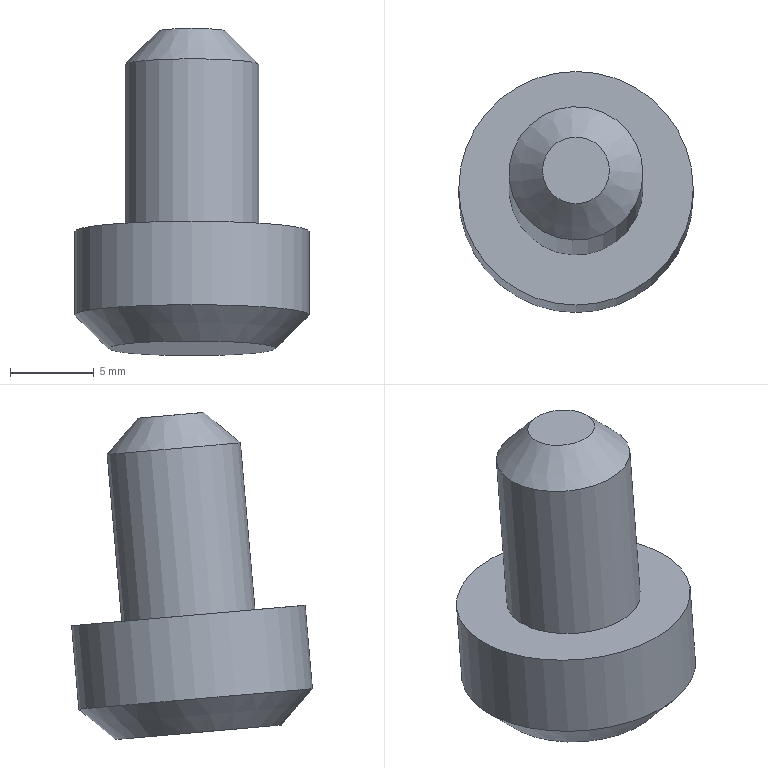Component | NX | BASE_FOOT | 1 solid | 7 faces | box 14 x 14.38 x 19.54 mm | volume 1559 mm3 | plane 3 | cylinder 2 | cone 2 | commonest cylinder face diameters 14 x1 8 x1
STEP:
#1=CARTESIAN_POINT('',(0.,0.,0.));
#2=DIRECTION('',(0.,0.,1.));
#3=DIRECTION('',(1.,0.,0.));
#4=AXIS2_PLACEMENT_3D('',#1,#2,#3);
#5=CARTESIAN_POINT('',(402.941,512.422,-69.71));
#6=VERTEX_POINT('',#5);
#7=CARTESIAN_POINT('',(395.941,512.422,-69.71));
#8=DIRECTION('',(0.,0.08716,0.9962));
#9=DIRECTION('',(1.,0.,0.));
#10=AXIS2_PLACEMENT_3D('',#7,#8,#9);
#11=CIRCLE('',#10,7.);
#12=CARTESIAN_POINT('',(395.941,512.858,-64.729));
#13=DIRECTION('',(0.,-0.08716,-0.9962));
#14=DIRECTION('',(-1.,0.,0.));
#15=AXIS2_PLACEMENT_3D('',#12,#13,#14);
#16=CYLINDRICAL_SURFACE('',#15,7.);
#17=CARTESIAN_POINT('',(9.425,5.));
#18=DIRECTION('',(-1.,0.));
#19=VECTOR('',#18,1.);
#20=LINE('',#17,#19);
#21=(GEOMETRIC_REPRESENTATION_CONTEXT(2)PARAMETRIC_REPRESENTATION_CONTEXT()REPRESENTATION_CONTEXT('',''));
#22=DEFINITIONAL_REPRESENTATION('',(#20),#21);
#23=PCURVE('',#16,#22);
#24=CARTESIAN_POINT('',(395.941,512.422,-69.71));
#25=DIRECTION('',(0.,0.08716,0.9962));
#26=DIRECTION('',(1.,0.,-0.));
#27=AXIS2_PLACEMENT_3D('',#24,#25,#26);
#28=CONICAL_SURFACE('',#27,7.,0.7854);
#29=CARTESIAN_POINT('',(0.,0.));
#30=DIRECTION('',(1.,0.));
#31=VECTOR('',#30,1.);
#32=LINE('',#29,#31);
#33=(GEOMETRIC_REPRESENTATION_CONTEXT(2)PARAMETRIC_REPRESENTATION_CONTEXT()REPRESENTATION_CONTEXT('',''));
#34=DEFINITIONAL_REPRESENTATION('',(#32),#33);
#35=PCURVE('',#28,#34);
#36=SURFACE_CURVE('',#11,(#23,#35),.PCURVE_S1.);
#37=EDGE_CURVE('',#6,#6,#36,.T.);
#38=ORIENTED_EDGE('',*,*,#37,.T.);
#39=CARTESIAN_POINT('',(402.941,512.858,-64.729));
#40=VERTEX_POINT('',#39);
#41=CARTESIAN_POINT('',(402.941,512.858,-64.729));
#42=CARTESIAN_POINT('',(402.941,512.422,-69.71));
#43=B_SPLINE_CURVE_WITH_KNOTS('',1,(#41,#42),.UNSPECIFIED.,.F.,.F.,(2,2),(0.,5.),.PIECEWISE_BEZIER_KNOTS.);
#44=CARTESIAN_POINT('',(3.142,0.));
#45=DIRECTION('',(0.,1.));
#46=VECTOR('',#45,1.);
#47=LINE('',#44,#46);
#48=(GEOMETRIC_REPRESENTATION_CONTEXT(2)PARAMETRIC_REPRESENTATION_CONTEXT()REPRESENTATION_CONTEXT('',''));
#49=DEFINITIONAL_REPRESENTATION('',(#47),#48);
#50=PCURVE('',#16,#49);
#51=CARTESIAN_POINT('',(9.425,0.));
#52=DIRECTION('',(0.,1.));
#53=VECTOR('',#52,1.);
#54=LINE('',#51,#53);
#55=(GEOMETRIC_REPRESENTATION_CONTEXT(2)PARAMETRIC_REPRESENTATION_CONTEXT()REPRESENTATION_CONTEXT('',''));
#56=DEFINITIONAL_REPRESENTATION('',(#54),#55);
#57=PCURVE('',#16,#56);
#58=SEAM_CURVE('',#43,(#50,#57),.PCURVE_S1.);
#59=EDGE_CURVE('',#40,#6,#58,.T.);
#60=ORIENTED_EDGE('',*,*,#59,.F.);
#61=CARTESIAN_POINT('',(395.941,512.858,-64.729));
#62=DIRECTION('',(0.,0.08716,0.9962));
#63=DIRECTION('',(1.,0.,0.));
#64=AXIS2_PLACEMENT_3D('',#61,#62,#63);
#65=CIRCLE('',#64,7.);
#66=CARTESIAN_POINT('',(9.425,0.));
#67=DIRECTION('',(-1.,0.));
#68=VECTOR('',#67,1.);
#69=LINE('',#66,#68);
#70=(GEOMETRIC_REPRESENTATION_CONTEXT(2)PARAMETRIC_REPRESENTATION_CONTEXT()REPRESENTATION_CONTEXT('',''));
#71=DEFINITIONAL_REPRESENTATION('',(#69),#70);
#72=PCURVE('',#16,#71);
#73=CARTESIAN_POINT('',(395.941,512.858,-64.729));
#74=DIRECTION('',(0.,0.08716,0.9962));
#75=DIRECTION('',(1.,0.,0.));
#76=AXIS2_PLACEMENT_3D('',#73,#74,#75);
#77=PLANE('',#76);
#78=CARTESIAN_POINT('',(0.,0.));
#79=DIRECTION('',(1.,0.));
#80=AXIS2_PLACEMENT_2D('',#78,#79);
#81=CIRCLE('',#80,7.);
#82=(GEOMETRIC_REPRESENTATION_CONTEXT(2)PARAMETRIC_REPRESENTATION_CONTEXT()REPRESENTATION_CONTEXT('',''));
#83=DEFINITIONAL_REPRESENTATION('',(#81),#82);
#84=PCURVE('',#77,#83);
#85=SURFACE_CURVE('',#65,(#72,#84),.PCURVE_S1.);
#86=EDGE_CURVE('',#40,#40,#85,.T.);
#87=ORIENTED_EDGE('',*,*,#86,.F.);
#88=ORIENTED_EDGE('',*,*,#59,.T.);
#89=EDGE_LOOP('',(#38,#60,#87,#88));
#90=FACE_BOUND('',#89,.T.);
#91=ADVANCED_FACE('',(#90),#16,.T.);
#92=CARTESIAN_POINT('',(399.941,512.858,-64.729));
#93=VERTEX_POINT('',#92);
#94=CARTESIAN_POINT('',(395.941,512.858,-64.729));
#95=DIRECTION('',(0.,0.08716,0.9962));
#96=DIRECTION('',(1.,0.,0.));
#97=AXIS2_PLACEMENT_3D('',#94,#95,#96);
#98=CIRCLE('',#97,4.);
#99=CARTESIAN_POINT('',(0.,0.));
#100=DIRECTION('',(1.,0.));
#101=AXIS2_PLACEMENT_2D('',#99,#100);
#102=CIRCLE('',#101,4.);
#103=(GEOMETRIC_REPRESENTATION_CONTEXT(2)PARAMETRIC_REPRESENTATION_CONTEXT()REPRESENTATION_CONTEXT('',''));
#104=DEFINITIONAL_REPRESENTATION('',(#102),#103);
#105=PCURVE('',#77,#104);
#106=CARTESIAN_POINT('',(395.941,513.904,-52.774));
#107=DIRECTION('',(0.,-0.08716,-0.9962));
#108=DIRECTION('',(-1.,0.,0.));
#109=AXIS2_PLACEMENT_3D('',#106,#107,#108);
#110=CYLINDRICAL_SURFACE('',#109,4.);
#111=CARTESIAN_POINT('',(9.425,12.));
#112=DIRECTION('',(-1.,0.));
#113=VECTOR('',#112,1.);
#114=LINE('',#111,#113);
#115=(GEOMETRIC_REPRESENTATION_CONTEXT(2)PARAMETRIC_REPRESENTATION_CONTEXT()REPRESENTATION_CONTEXT('',''));
#116=DEFINITIONAL_REPRESENTATION('',(#114),#115);
#117=PCURVE('',#110,#116);
#118=SURFACE_CURVE('',#98,(#105,#117),.PCURVE_S1.);
#119=EDGE_CURVE('',#93,#93,#118,.T.);
#120=ORIENTED_EDGE('',*,*,#119,.F.);
#121=EDGE_LOOP('',(#120));
#122=FACE_BOUND('',#121,.T.);
#123=ORIENTED_EDGE('',*,*,#86,.T.);
#124=EDGE_LOOP('',(#123));
#125=FACE_BOUND('',#124,.T.);
#126=ADVANCED_FACE('',(#122,#125),#77,.T.);
#127=CARTESIAN_POINT('',(400.941,512.248,-71.702));
#128=VERTEX_POINT('',#127);
#129=CARTESIAN_POINT('',(395.941,512.248,-71.702));
#130=DIRECTION('',(0.,-0.08716,-0.9962));
#131=DIRECTION('',(1.,0.,0.));
#132=AXIS2_PLACEMENT_3D('',#129,#130,#131);
#133=CIRCLE('',#132,5.);
#134=CARTESIAN_POINT('',(395.941,512.248,-71.702));
#135=DIRECTION('',(0.,0.08716,0.9962));
#136=DIRECTION('',(1.,0.,0.));
#137=AXIS2_PLACEMENT_3D('',#134,#135,#136);
#138=PLANE('',#137);
#139=CARTESIAN_POINT('',(5.,0.));
#140=CARTESIAN_POINT('',(5.,-8.66));
#141=CARTESIAN_POINT('',(-2.5,-4.33));
#142=CARTESIAN_POINT('',(-10.,-0.));
#143=CARTESIAN_POINT('',(-2.5,4.33));
#144=CARTESIAN_POINT('',(5.,8.66));
#145=CARTESIAN_POINT('',(5.,0.));
#146=(BOUNDED_CURVE()B_SPLINE_CURVE(2,(#139,#140,#141,#142,#143,#144,#145),.UNSPECIFIED.,.T.,.F.)B_SPLINE_CURVE_WITH_KNOTS((1,2,2,2,2,1),(-2.094,0.,2.094,4.189,6.283,8.378),.UNSPECIFIED.)CURVE()GEOMETRIC_REPRESENTATION_ITEM()RATIONAL_B_SPLINE_CURVE((1.,0.5,1.,0.5,1.,0.5,1.))REPRESENTATION_ITEM(''));
#147=(GEOMETRIC_REPRESENTATION_CONTEXT(2)PARAMETRIC_REPRESENTATION_CONTEXT()REPRESENTATION_CONTEXT('',''));
#148=DEFINITIONAL_REPRESENTATION('',(#146),#147);
#149=PCURVE('',#138,#148);
#150=CARTESIAN_POINT('',(6.283,-2.));
#151=DIRECTION('',(-1.,0.));
#152=VECTOR('',#151,1.);
#153=LINE('',#150,#152);
#154=(GEOMETRIC_REPRESENTATION_CONTEXT(2)PARAMETRIC_REPRESENTATION_CONTEXT()REPRESENTATION_CONTEXT('',''));
#155=DEFINITIONAL_REPRESENTATION('',(#153),#154);
#156=PCURVE('',#28,#155);
#157=SURFACE_CURVE('',#133,(#149,#156),.PCURVE_S1.);
#158=EDGE_CURVE('',#128,#128,#157,.T.);
#159=ORIENTED_EDGE('',*,*,#158,.T.);
#160=EDGE_LOOP('',(#159));
#161=FACE_BOUND('',#160,.T.);
#162=ADVANCED_FACE('',(#161),#138,.F.);
#163=CARTESIAN_POINT('',(399.941,513.729,-54.767));
#164=VERTEX_POINT('',#163);
#165=CARTESIAN_POINT('',(395.941,513.729,-54.767));
#166=DIRECTION('',(0.,-0.08716,-0.9962));
#167=DIRECTION('',(1.,0.,0.));
#168=AXIS2_PLACEMENT_3D('',#165,#166,#167);
#169=CIRCLE('',#168,4.);
#170=CARTESIAN_POINT('',(3.142,2.));
#171=DIRECTION('',(1.,0.));
#172=VECTOR('',#171,1.);
#173=LINE('',#170,#172);
#174=(GEOMETRIC_REPRESENTATION_CONTEXT(2)PARAMETRIC_REPRESENTATION_CONTEXT()REPRESENTATION_CONTEXT('',''));
#175=DEFINITIONAL_REPRESENTATION('',(#173),#174);
#176=PCURVE('',#110,#175);
#177=CARTESIAN_POINT('',(395.941,513.904,-52.774));
#178=DIRECTION('',(0.,-0.08716,-0.9962));
#179=DIRECTION('',(-1.,-0.,0.));
#180=AXIS2_PLACEMENT_3D('',#177,#178,#179);
#181=CONICAL_SURFACE('',#180,2.,0.7854);
#182=CARTESIAN_POINT('',(3.142,2.));
#183=DIRECTION('',(1.,0.));
#184=VECTOR('',#183,1.);
#185=LINE('',#182,#184);
#186=(GEOMETRIC_REPRESENTATION_CONTEXT(2)PARAMETRIC_REPRESENTATION_CONTEXT()REPRESENTATION_CONTEXT('',''));
#187=DEFINITIONAL_REPRESENTATION('',(#185),#186);
#188=PCURVE('',#181,#187);
#189=SURFACE_CURVE('',#169,(#176,#188),.PCURVE_S1.);
#190=EDGE_CURVE('',#164,#164,#189,.T.);
#191=ORIENTED_EDGE('',*,*,#190,.T.);
#192=CARTESIAN_POINT('',(399.941,513.729,-54.767));
#193=CARTESIAN_POINT('',(399.941,512.858,-64.729));
#194=B_SPLINE_CURVE_WITH_KNOTS('',1,(#192,#193),.UNSPECIFIED.,.F.,.F.,(2,2),(2.,12.),.PIECEWISE_BEZIER_KNOTS.);
#195=CARTESIAN_POINT('',(9.425,0.));
#196=DIRECTION('',(0.,1.));
#197=VECTOR('',#196,1.);
#198=LINE('',#195,#197);
#199=(GEOMETRIC_REPRESENTATION_CONTEXT(2)PARAMETRIC_REPRESENTATION_CONTEXT()REPRESENTATION_CONTEXT('',''));
#200=DEFINITIONAL_REPRESENTATION('',(#198),#199);
#201=PCURVE('',#110,#200);
#202=CARTESIAN_POINT('',(3.142,0.));
#203=DIRECTION('',(0.,1.));
#204=VECTOR('',#203,1.);
#205=LINE('',#202,#204);
#206=(GEOMETRIC_REPRESENTATION_CONTEXT(2)PARAMETRIC_REPRESENTATION_CONTEXT()REPRESENTATION_CONTEXT('',''));
#207=DEFINITIONAL_REPRESENTATION('',(#205),#206);
#208=PCURVE('',#110,#207);
#209=SEAM_CURVE('',#194,(#201,#208),.PCURVE_S1.);
#210=EDGE_CURVE('',#164,#93,#209,.T.);
#211=ORIENTED_EDGE('',*,*,#210,.T.);
#212=ORIENTED_EDGE('',*,*,#119,.T.);
#213=ORIENTED_EDGE('',*,*,#210,.F.);
#214=EDGE_LOOP('',(#191,#211,#212,#213));
#215=FACE_BOUND('',#214,.T.);
#216=ADVANCED_FACE('',(#215),#110,.T.);
#217=CARTESIAN_POINT('',(397.941,513.904,-52.774));
#218=VERTEX_POINT('',#217);
#219=CARTESIAN_POINT('',(395.941,513.904,-52.774));
#220=DIRECTION('',(0.,0.08716,0.9962));
#221=DIRECTION('',(1.,0.,0.));
#222=AXIS2_PLACEMENT_3D('',#219,#220,#221);
#223=CIRCLE('',#222,2.);
#224=CARTESIAN_POINT('',(395.941,513.904,-52.774));
#225=DIRECTION('',(0.,0.08716,0.9962));
#226=DIRECTION('',(1.,0.,0.));
#227=AXIS2_PLACEMENT_3D('',#224,#225,#226);
#228=PLANE('',#227);
#229=CARTESIAN_POINT('',(0.,0.));
#230=DIRECTION('',(1.,0.));
#231=AXIS2_PLACEMENT_2D('',#229,#230);
#232=CIRCLE('',#231,2.);
#233=(GEOMETRIC_REPRESENTATION_CONTEXT(2)PARAMETRIC_REPRESENTATION_CONTEXT()REPRESENTATION_CONTEXT('',''));
#234=DEFINITIONAL_REPRESENTATION('',(#232),#233);
#235=PCURVE('',#228,#234);
#236=CARTESIAN_POINT('',(9.425,0.));
#237=DIRECTION('',(-1.,0.));
#238=VECTOR('',#237,1.);
#239=LINE('',#236,#238);
#240=(GEOMETRIC_REPRESENTATION_CONTEXT(2)PARAMETRIC_REPRESENTATION_CONTEXT()REPRESENTATION_CONTEXT('',''));
#241=DEFINITIONAL_REPRESENTATION('',(#239),#240);
#242=PCURVE('',#181,#241);
#243=SURFACE_CURVE('',#223,(#235,#242),.PCURVE_S1.);
#244=EDGE_CURVE('',#218,#218,#243,.T.);
#245=ORIENTED_EDGE('',*,*,#244,.T.);
#246=EDGE_LOOP('',(#245));
#247=FACE_BOUND('',#246,.T.);
#248=ADVANCED_FACE('',(#247),#228,.T.);
#249=ORIENTED_EDGE('',*,*,#158,.F.);
#250=CARTESIAN_POINT('',(400.941,512.248,-71.702));
#251=CARTESIAN_POINT('',(402.941,512.422,-69.71));
#252=B_SPLINE_CURVE_WITH_KNOTS('',1,(#250,#251),.UNSPECIFIED.,.F.,.F.,(2,2),(-2.828,0.),.PIECEWISE_BEZIER_KNOTS.);
#253=CARTESIAN_POINT('',(6.283,0.));
#254=DIRECTION('',(0.,1.));
#255=VECTOR('',#254,1.);
#256=LINE('',#253,#255);
#257=(GEOMETRIC_REPRESENTATION_CONTEXT(2)PARAMETRIC_REPRESENTATION_CONTEXT()REPRESENTATION_CONTEXT('',''));
#258=DEFINITIONAL_REPRESENTATION('',(#256),#257);
#259=PCURVE('',#28,#258);
#260=CARTESIAN_POINT('',(0.,0.));
#261=DIRECTION('',(0.,1.));
#262=VECTOR('',#261,1.);
#263=LINE('',#260,#262);
#264=(GEOMETRIC_REPRESENTATION_CONTEXT(2)PARAMETRIC_REPRESENTATION_CONTEXT()REPRESENTATION_CONTEXT('',''));
#265=DEFINITIONAL_REPRESENTATION('',(#263),#264);
#266=PCURVE('',#28,#265);
#267=SEAM_CURVE('',#252,(#259,#266),.PCURVE_S1.);
#268=EDGE_CURVE('',#128,#6,#267,.T.);
#269=ORIENTED_EDGE('',*,*,#268,.T.);
#270=ORIENTED_EDGE('',*,*,#37,.F.);
#271=ORIENTED_EDGE('',*,*,#268,.F.);
#272=EDGE_LOOP('',(#249,#269,#270,#271));
#273=FACE_BOUND('',#272,.T.);
#274=ADVANCED_FACE('',(#273),#28,.T.);
#275=ORIENTED_EDGE('',*,*,#190,.F.);
#276=CARTESIAN_POINT('',(397.941,513.904,-52.774));
#277=CARTESIAN_POINT('',(399.941,513.729,-54.767));
#278=B_SPLINE_CURVE_WITH_KNOTS('',1,(#276,#277),.UNSPECIFIED.,.F.,.F.,(2,2),(0.,2.828),.PIECEWISE_BEZIER_KNOTS.);
#279=CARTESIAN_POINT('',(3.142,0.));
#280=DIRECTION('',(0.,1.));
#281=VECTOR('',#280,1.);
#282=LINE('',#279,#281);
#283=(GEOMETRIC_REPRESENTATION_CONTEXT(2)PARAMETRIC_REPRESENTATION_CONTEXT()REPRESENTATION_CONTEXT('',''));
#284=DEFINITIONAL_REPRESENTATION('',(#282),#283);
#285=PCURVE('',#181,#284);
#286=CARTESIAN_POINT('',(9.425,0.));
#287=DIRECTION('',(0.,1.));
#288=VECTOR('',#287,1.);
#289=LINE('',#286,#288);
#290=(GEOMETRIC_REPRESENTATION_CONTEXT(2)PARAMETRIC_REPRESENTATION_CONTEXT()REPRESENTATION_CONTEXT('',''));
#291=DEFINITIONAL_REPRESENTATION('',(#289),#290);
#292=PCURVE('',#181,#291);
#293=SEAM_CURVE('',#278,(#285,#292),.PCURVE_S1.);
#294=EDGE_CURVE('',#218,#164,#293,.T.);
#295=ORIENTED_EDGE('',*,*,#294,.F.);
#296=ORIENTED_EDGE('',*,*,#244,.F.);
#297=ORIENTED_EDGE('',*,*,#294,.T.);
#298=EDGE_LOOP('',(#275,#295,#296,#297));
#299=FACE_BOUND('',#298,.T.);
#300=ADVANCED_FACE('',(#299),#181,.T.);
#301=CLOSED_SHELL('',(#91,#126,#162,#216,#248,#274,#300));
#302=MANIFOLD_SOLID_BREP('',#301);
#303=(LENGTH_UNIT()NAMED_UNIT(*)SI_UNIT(.MILLI.,.METRE.));
#304=UNCERTAINTY_MEASURE_WITH_UNIT(LENGTH_MEASURE(0.00001),#303,'','');
#305=(NAMED_UNIT(*)PLANE_ANGLE_UNIT()SI_UNIT($,.RADIAN.));
#306=(NAMED_UNIT(*)SI_UNIT($,.STERADIAN.)SOLID_ANGLE_UNIT());
#307=(GEOMETRIC_REPRESENTATION_CONTEXT(3)GLOBAL_UNCERTAINTY_ASSIGNED_CONTEXT((#304))GLOBAL_UNIT_ASSIGNED_CONTEXT((#303,#305,#306))REPRESENTATION_CONTEXT('',''));
#308=ADVANCED_BREP_SHAPE_REPRESENTATION('',(#4,#302),#307);